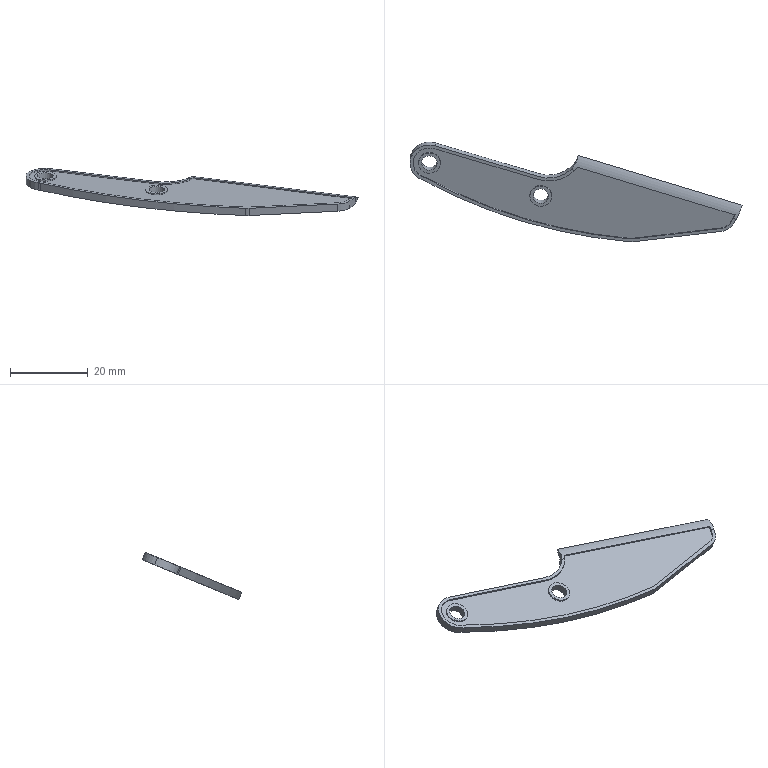Component | SolidWorks | MirrorThe Claw-2 | 1 solid | 55 faces | volume 1496 mm3 | cylinder 34 | plane 21 | commonest cylinder face diameters 5.6 x8 4 x4 6.4 x4 8.4 x3 8 x3 16 x3 10 x2 9.6 x2